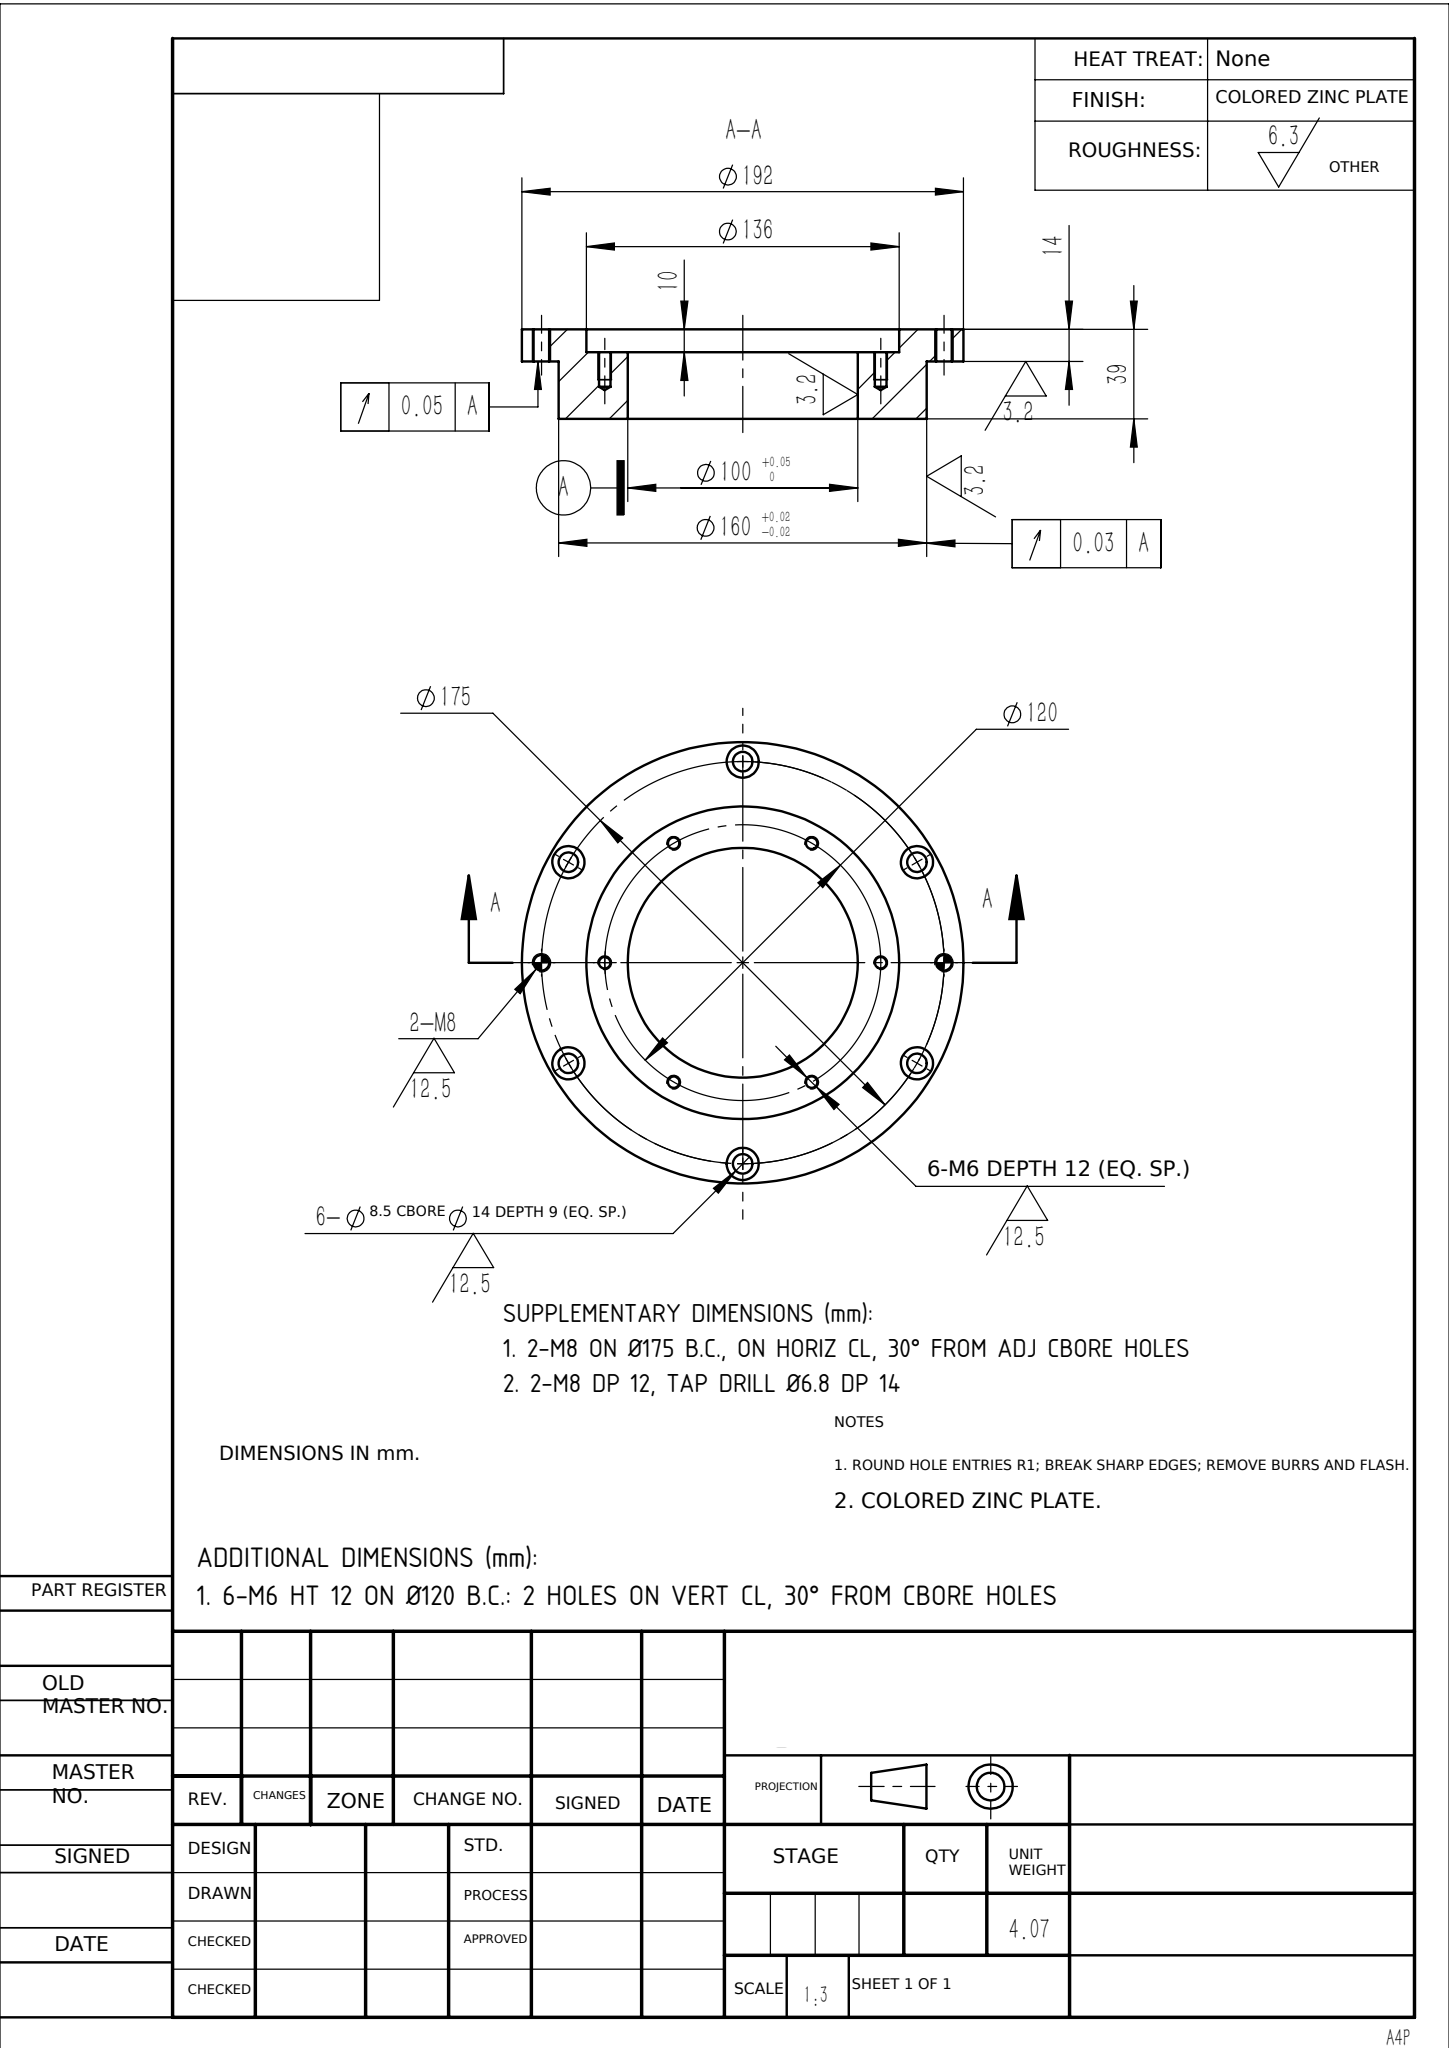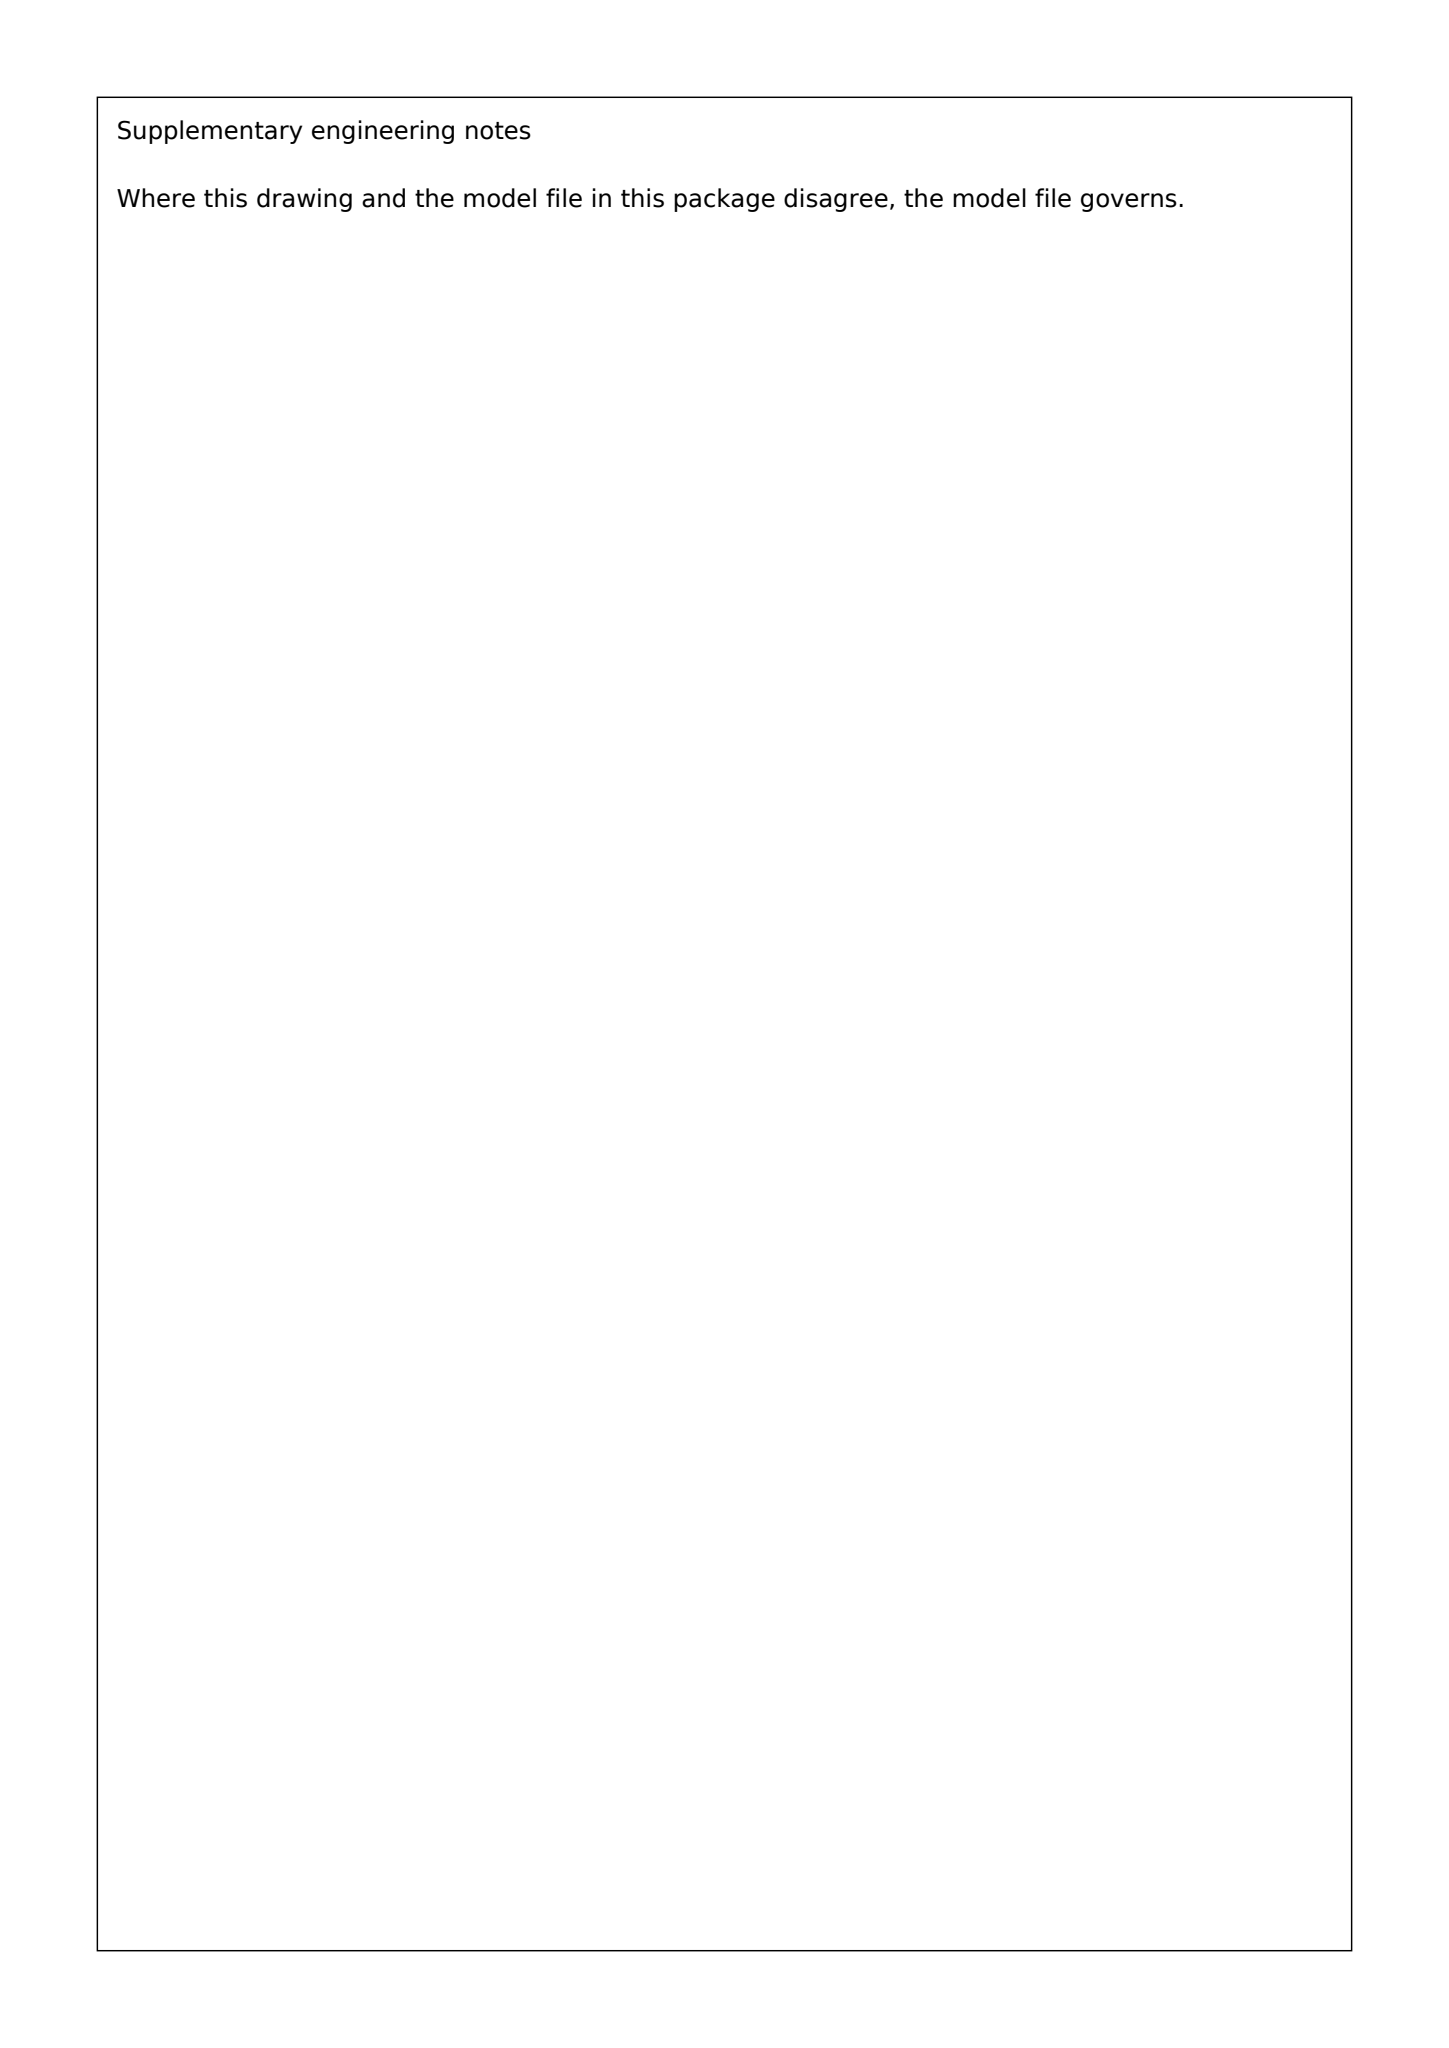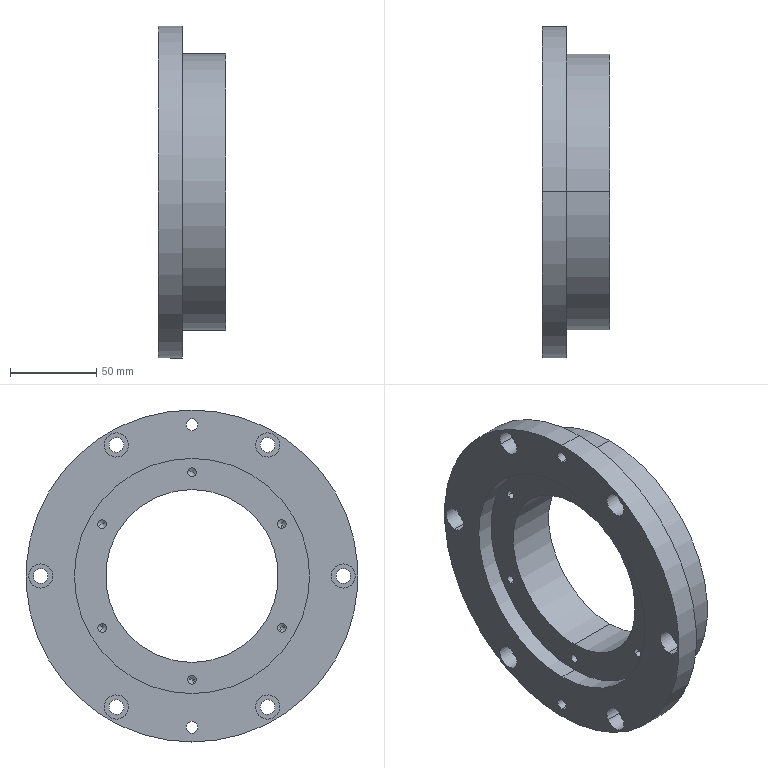Part | SolidWorks | mm | 1 solid | 70 faces | box 39 x 192 x 192 mm | volume 522105 mm3 | cylinder 48 | cone 12 | plane 10 | commonest cylinder face diameters 5 x12 14 x12 8.5 x12 6.8 x4 136 x2 192 x2 160 x2 100 x2
build123d program:
from build123d import *

# Parameters (mm, degrees)
SKETCH3_R          = 4.25
CUT_EXTRUDE1_DEPTH = 139.047
M8_TAPPED_HOLE1_D  = 6.8
SKETCH10_R         = 68
CUT_EXTRUDE3_DEPTH = 10
SKETCH9_R          = 7
CUT_EXTRUDE2_DEPTH = 9
CIRPATTERN1_COUNT  = 6
CIRPATTERN2_COUNT  = 6


with BuildPart() as part:
    # Sketch2 → Revolve1 (revolve)
    with BuildSketch(Plane.XY, mode=Mode.PRIVATE) as revolve1_sk:
        Polygon((0, 50), (0, 96), (14, 96), (14, 80), (39, 80), (39, 50), align=None)
    revolve(revolve1_sk.sketch.rotate(Axis((0, 0, 0), (1, 0, 0)), 90), axis=Axis((0, 0, 0), (1, 0, 0)))

    # Sketch3 → Cut-Extrude1 (cut, through all)
    with BuildSketch(Plane(origin=(14, 0, 0), x_dir=(0, 0, -1), z_dir=(1, 0, 0))):
        with Locations((0, 87.5)):
            Circle(SKETCH3_R)
    cut_extrude1 = extrude(amount=-CUT_EXTRUDE1_DEPTH, mode=Mode.SUBTRACT)

    # M8 Tapped Hole1 (through all)
    with Locations(Plane.ZY):
        with Locations((-87.5, 0), (87.5, 0)):
            Hole(M8_TAPPED_HOLE1_D / 2)

    # Sketch10 → Cut-Extrude3 (cut)
    with BuildSketch(Plane.ZY):
        Circle(SKETCH10_R)
    extrude(amount=-CUT_EXTRUDE3_DEPTH, mode=Mode.SUBTRACT)

    # Sketch8 → M6 Tapped Hole1 (revolve, cut)
    with BuildSketch(Plane(origin=(10, 51.962, -30), x_dir=(0, 0, 1), z_dir=(0, 1, 0))):
        Polygon((0, 0), (0, 16.502), (2.5, 15), (2.5, 0), align=None)
    m6_tapped_hole1 = revolve(axis=Axis((3.65, 51.962, -30), (1, 0, 0)), mode=Mode.SUBTRACT)

    # Sketch9 → Cut-Extrude2 (cut)
    with BuildSketch(Plane.ZY):
        with Locations((0, 87.5)):
            Circle(SKETCH9_R)
    cut_extrude2 = extrude(amount=-CUT_EXTRUDE2_DEPTH, mode=Mode.SUBTRACT)

    # CirPattern1: Cut-Extrude1, Cut-Extrude2 ×6 about axis
    cirpattern1_axis = Axis((0, 0, 0), (1, 0, 0))
    add([cut_extrude1.rotate(cirpattern1_axis, i * 360 / CIRPATTERN1_COUNT) for i in range(1, CIRPATTERN1_COUNT)], mode=Mode.SUBTRACT)
    add([cut_extrude2.rotate(cirpattern1_axis, i * 360 / CIRPATTERN1_COUNT) for i in range(1, CIRPATTERN1_COUNT)], mode=Mode.SUBTRACT)

    # CirPattern2: M6 Tapped Hole1 ×6 about axis
    cirpattern2_axis = Axis((0, 0, 0), (1, 0, 0))
    for i in range(1, CIRPATTERN2_COUNT):
        add(m6_tapped_hole1.rotate(cirpattern2_axis, i * 360 / CIRPATTERN2_COUNT), mode=Mode.SUBTRACT)


solid = part.part